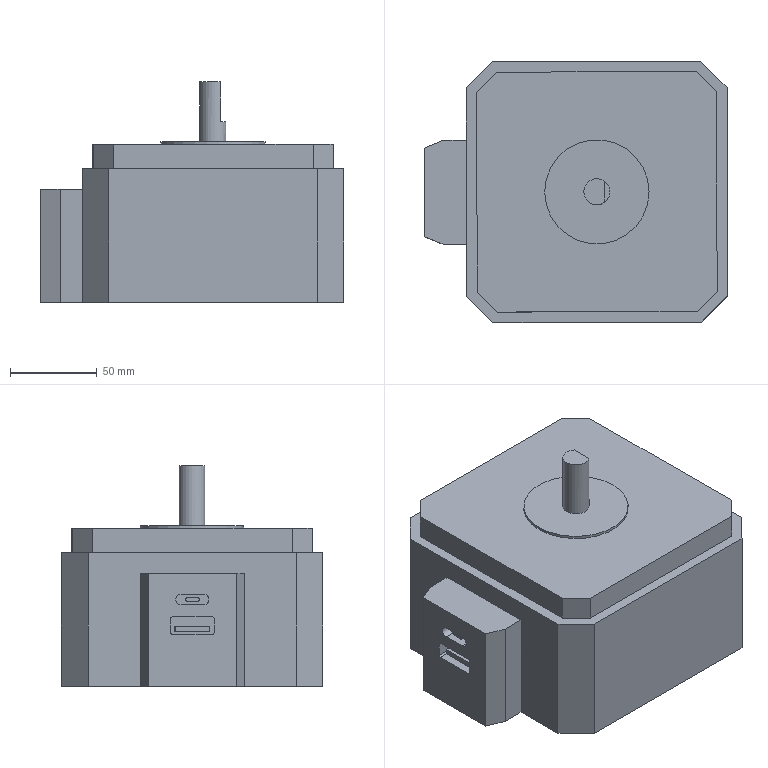Component | NX | INTEGRATED_STEPPER_MOTOR | 1 solid | 55 faces | volume 2057190 mm3 | plane 45 | cylinder 10 | commonest cylinder face diameters 2 x6 6 x2 60 x1 15 x1